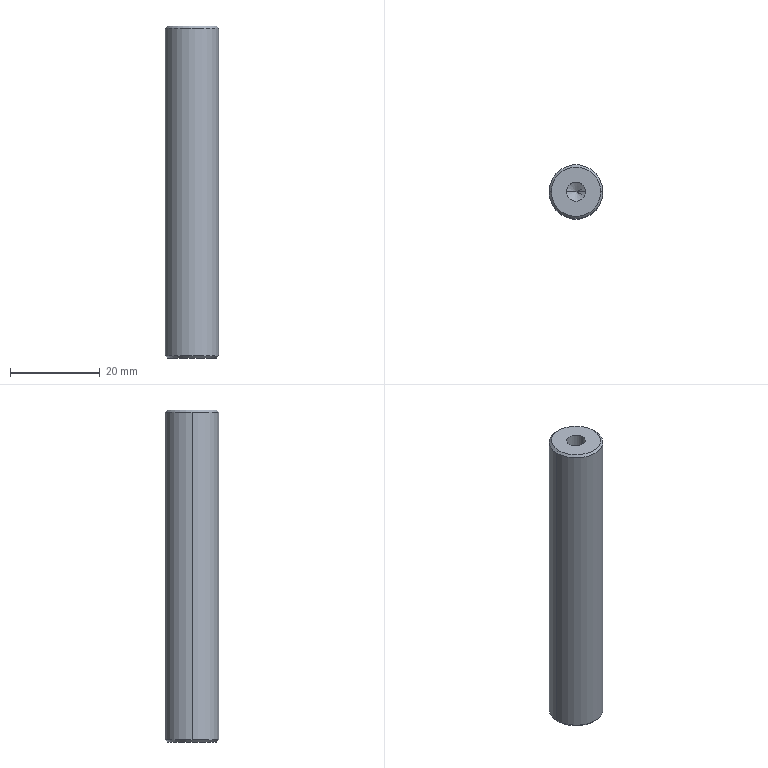Component | SolidWorks | J-028-1 | 1 solid | 12 faces | box 12 x 12 x 74 mm | volume 8182 mm3 | cone 6 | cylinder 4 | plane 2 | commonest cylinder face diameters 4.2 x2 12 x2 | material 45
build123d program:
from build123d import *

# Parameters (mm, degrees)
SKETCH1_R             = 6
BOSS_EXTRUDE1_DEPTH   = 74
CHAMFER1_SIZE         = 0.5
M5_TAPPED_HOLE1_D     = 4.2
M5_TAPPED_HOLE1_DEPTH = 12.4
M5_TAPPED_HOLE1_TIP   = 1.262


with BuildPart() as part:
    # Sketch1 → Boss-Extrude1 (new body)
    with BuildSketch(Plane(origin=(0, 0, 0), x_dir=(0, 0, -1), z_dir=(1, 0, 0))):
        Circle(SKETCH1_R)
    extrude(amount=BOSS_EXTRUDE1_DEPTH)

    # Chamfer1
    chamfer1_edges = [part.edges().sort_by_distance(p)[0] for p in [
        (0, 0, 6),
        (74, 0, 6),
    ]]
    chamfer(chamfer1_edges, length=CHAMFER1_SIZE)

    # M5 Tapped Hole1
    with Locations(Plane.ZY):
        with Locations((0, 0)):
            Hole(M5_TAPPED_HOLE1_D / 2, depth=M5_TAPPED_HOLE1_DEPTH)
            with Locations((0, 0, -(M5_TAPPED_HOLE1_DEPTH + M5_TAPPED_HOLE1_TIP / 2))):  # 118° drill point
                Cone(0, M5_TAPPED_HOLE1_D / 2, M5_TAPPED_HOLE1_TIP, mode=Mode.SUBTRACT)


solid = part.part

# Placed as in the assembly
solid = solid.moved(Location((95.325, 243.019, 264.731), (0, 90, 0)))
STEP:
#1=COLOUR_RGB('',0.7922,0.8196,0.9333);
#2=FILL_AREA_STYLE_COLOUR('',#1);
#3=FILL_AREA_STYLE('',(#2));
#4=SURFACE_STYLE_FILL_AREA(#3);
#5=SURFACE_SIDE_STYLE('',(#4));
#6=SURFACE_STYLE_USAGE(.BOTH.,#5);
#7=PRESENTATION_STYLE_ASSIGNMENT((#6));
#8=CARTESIAN_POINT('',(3.67,9.568,9.934));
#9=VERTEX_POINT('',#8);
#10=CARTESIAN_POINT('',(3.836,9.568,9.934));
#11=VERTEX_POINT('',#10);
#12=CARTESIAN_POINT('',(3.753,9.568,9.934));
#13=DIRECTION('',(0.,0.,1.));
#14=DIRECTION('',(1.,0.,0.));
#15=AXIS2_PLACEMENT_3D('',#12,#13,#14);
#16=CIRCLE('',#15,0.08268);
#17=EDGE_CURVE('',#9,#11,#16,.T.);
#18=ORIENTED_EDGE('',*,*,#17,.F.);
#19=CARTESIAN_POINT('',(3.67,9.568,10.422));
#20=VERTEX_POINT('',#19);
#21=CARTESIAN_POINT('',(3.67,9.568,10.422));
#22=DIRECTION('',(0.,0.,1.));
#23=VECTOR('',#22,39.37);
#24=LINE('',#21,#23);
#25=EDGE_CURVE('',#9,#20,#24,.T.);
#26=ORIENTED_EDGE('',*,*,#25,.T.);
#27=CARTESIAN_POINT('',(3.836,9.568,10.422));
#28=VERTEX_POINT('',#27);
#29=CARTESIAN_POINT('',(3.753,9.568,10.422));
#30=DIRECTION('',(0.,0.,1.));
#31=DIRECTION('',(1.,0.,0.));
#32=AXIS2_PLACEMENT_3D('',#29,#30,#31);
#33=CIRCLE('',#32,0.08268);
#34=EDGE_CURVE('',#20,#28,#33,.T.);
#35=ORIENTED_EDGE('',*,*,#34,.T.);
#36=CARTESIAN_POINT('',(3.836,9.568,10.422));
#37=DIRECTION('',(0.,0.,1.));
#38=VECTOR('',#37,39.37);
#39=LINE('',#36,#38);
#40=EDGE_CURVE('',#11,#28,#39,.T.);
#41=ORIENTED_EDGE('',*,*,#40,.F.);
#42=EDGE_LOOP('',(#18,#26,#35,#41));
#43=FACE_OUTER_BOUND('',#42,.T.);
#44=CARTESIAN_POINT('',(3.753,9.568,10.422));
#45=DIRECTION('',(0.,0.,1.));
#46=DIRECTION('',(1.,0.,0.));
#47=AXIS2_PLACEMENT_3D('',#44,#45,#46);
#48=CYLINDRICAL_SURFACE('',#47,0.08268);
#49=ADVANCED_FACE('',(#43),#48,.F.);
#50=CARTESIAN_POINT('',(3.753,9.568,9.885));
#51=VERTEX_POINT('',#50);
#52=CARTESIAN_POINT('',(3.836,9.568,9.934));
#53=DIRECTION('',(0.8572,0.,0.515));
#54=VECTOR('',#53,39.37);
#55=LINE('',#52,#54);
#56=EDGE_CURVE('',#51,#11,#55,.T.);
#57=ORIENTED_EDGE('',*,*,#56,.F.);
#58=CARTESIAN_POINT('',(3.67,9.568,9.934));
#59=DIRECTION('',(-0.8572,0.,0.515));
#60=VECTOR('',#59,39.37);
#61=LINE('',#58,#60);
#62=EDGE_CURVE('',#51,#9,#61,.T.);
#63=ORIENTED_EDGE('',*,*,#62,.T.);
#64=ORIENTED_EDGE('',*,*,#17,.T.);
#65=EDGE_LOOP('',(#57,#63,#64));
#66=FACE_OUTER_BOUND('',#65,.T.);
#67=CARTESIAN_POINT('',(3.753,9.568,9.934));
#68=DIRECTION('',(0.,0.,1.));
#69=DIRECTION('',(1.,0.,0.));
#70=AXIS2_PLACEMENT_3D('',#67,#68,#69);
#71=CONICAL_SURFACE('',#70,0.08268,1.03);
#72=ADVANCED_FACE('',(#66),#71,.F.);
#73=CARTESIAN_POINT('',(3.969,9.568,10.422));
#74=VERTEX_POINT('',#73);
#75=CARTESIAN_POINT('',(3.536,9.568,10.422));
#76=VERTEX_POINT('',#75);
#77=CARTESIAN_POINT('',(3.753,9.568,10.422));
#78=DIRECTION('',(0.,0.,1.));
#79=DIRECTION('',(-1.,0.,0.));
#80=AXIS2_PLACEMENT_3D('',#77,#78,#79);
#81=CIRCLE('',#80,0.2165);
#82=EDGE_CURVE('',#74,#76,#81,.T.);
#83=ORIENTED_EDGE('',*,*,#82,.F.);
#84=CARTESIAN_POINT('',(3.989,9.568,10.403));
#85=VERTEX_POINT('',#84);
#86=CARTESIAN_POINT('',(3.989,9.568,10.403));
#87=DIRECTION('',(0.7071,0.,-0.7071));
#88=VECTOR('',#87,39.37);
#89=LINE('',#86,#88);
#90=EDGE_CURVE('',#74,#85,#89,.T.);
#91=ORIENTED_EDGE('',*,*,#90,.T.);
#92=CARTESIAN_POINT('',(3.517,9.568,10.403));
#93=VERTEX_POINT('',#92);
#94=CARTESIAN_POINT('',(3.753,9.568,10.403));
#95=DIRECTION('',(0.,0.,-1.));
#96=DIRECTION('',(-1.,0.,0.));
#97=AXIS2_PLACEMENT_3D('',#94,#95,#96);
#98=CIRCLE('',#97,0.2362);
#99=EDGE_CURVE('',#93,#85,#98,.T.);
#100=ORIENTED_EDGE('',*,*,#99,.F.);
#101=CARTESIAN_POINT('',(3.517,9.568,10.403));
#102=DIRECTION('',(-0.7071,0.,-0.7071));
#103=VECTOR('',#102,39.37);
#104=LINE('',#101,#103);
#105=EDGE_CURVE('',#76,#93,#104,.T.);
#106=ORIENTED_EDGE('',*,*,#105,.F.);
#107=EDGE_LOOP('',(#83,#91,#100,#106));
#108=FACE_OUTER_BOUND('',#107,.T.);
#109=CARTESIAN_POINT('',(3.753,9.568,10.403));
#110=DIRECTION('',(0.,0.,-1.));
#111=DIRECTION('',(-1.,0.,0.));
#112=AXIS2_PLACEMENT_3D('',#109,#110,#111);
#113=CONICAL_SURFACE('',#112,0.2362,0.7854);
#114=ADVANCED_FACE('',(#108),#113,.T.);
#115=CARTESIAN_POINT('',(3.536,9.568,7.509));
#116=VERTEX_POINT('',#115);
#117=CARTESIAN_POINT('',(3.969,9.568,7.509));
#118=VERTEX_POINT('',#117);
#119=CARTESIAN_POINT('',(3.753,9.568,7.509));
#120=DIRECTION('',(0.,0.,-1.));
#121=DIRECTION('',(-1.,0.,0.));
#122=AXIS2_PLACEMENT_3D('',#119,#120,#121);
#123=CIRCLE('',#122,0.2165);
#124=EDGE_CURVE('',#116,#118,#123,.T.);
#125=ORIENTED_EDGE('',*,*,#124,.F.);
#126=CARTESIAN_POINT('',(3.517,9.568,7.529));
#127=VERTEX_POINT('',#126);
#128=CARTESIAN_POINT('',(3.536,9.568,7.509));
#129=DIRECTION('',(-0.7071,0.,0.7071));
#130=VECTOR('',#129,39.37);
#131=LINE('',#128,#130);
#132=EDGE_CURVE('',#116,#127,#131,.T.);
#133=ORIENTED_EDGE('',*,*,#132,.T.);
#134=CARTESIAN_POINT('',(3.989,9.568,7.529));
#135=VERTEX_POINT('',#134);
#136=CARTESIAN_POINT('',(3.753,9.568,7.529));
#137=DIRECTION('',(0.,0.,1.));
#138=DIRECTION('',(-1.,0.,0.));
#139=AXIS2_PLACEMENT_3D('',#136,#137,#138);
#140=CIRCLE('',#139,0.2362);
#141=EDGE_CURVE('',#135,#127,#140,.T.);
#142=ORIENTED_EDGE('',*,*,#141,.F.);
#143=CARTESIAN_POINT('',(3.969,9.568,7.509));
#144=DIRECTION('',(0.7071,0.,0.7071));
#145=VECTOR('',#144,39.37);
#146=LINE('',#143,#145);
#147=EDGE_CURVE('',#118,#135,#146,.T.);
#148=ORIENTED_EDGE('',*,*,#147,.F.);
#149=EDGE_LOOP('',(#125,#133,#142,#148));
#150=FACE_OUTER_BOUND('',#149,.T.);
#151=CARTESIAN_POINT('',(3.753,9.568,7.509));
#152=DIRECTION('',(0.,0.,1.));
#153=DIRECTION('',(1.,0.,0.));
#154=AXIS2_PLACEMENT_3D('',#151,#152,#153);
#155=CONICAL_SURFACE('',#154,0.2165,0.7854);
#156=ADVANCED_FACE('',(#150),#155,.T.);
#157=ORIENTED_EDGE('',*,*,#141,.T.);
#158=CARTESIAN_POINT('',(3.517,9.568,7.509));
#159=DIRECTION('',(0.,0.,1.));
#160=VECTOR('',#159,39.37);
#161=LINE('',#158,#160);
#162=EDGE_CURVE('',#127,#93,#161,.T.);
#163=ORIENTED_EDGE('',*,*,#162,.T.);
#164=ORIENTED_EDGE('',*,*,#99,.T.);
#165=CARTESIAN_POINT('',(3.989,9.568,7.509));
#166=DIRECTION('',(0.,0.,1.));
#167=VECTOR('',#166,39.37);
#168=LINE('',#165,#167);
#169=EDGE_CURVE('',#135,#85,#168,.T.);
#170=ORIENTED_EDGE('',*,*,#169,.F.);
#171=EDGE_LOOP('',(#157,#163,#164,#170));
#172=FACE_OUTER_BOUND('',#171,.T.);
#173=CARTESIAN_POINT('',(3.753,9.568,7.509));
#174=DIRECTION('',(0.,0.,1.));
#175=DIRECTION('',(1.,0.,0.));
#176=AXIS2_PLACEMENT_3D('',#173,#174,#175);
#177=CYLINDRICAL_SURFACE('',#176,0.2362);
#178=ADVANCED_FACE('',(#172),#177,.T.);
#179=ORIENTED_EDGE('',*,*,#162,.F.);
#180=CARTESIAN_POINT('',(3.753,9.568,7.529));
#181=DIRECTION('',(0.,0.,1.));
#182=DIRECTION('',(-1.,0.,0.));
#183=AXIS2_PLACEMENT_3D('',#180,#181,#182);
#184=CIRCLE('',#183,0.2362);
#185=EDGE_CURVE('',#127,#135,#184,.T.);
#186=ORIENTED_EDGE('',*,*,#185,.T.);
#187=ORIENTED_EDGE('',*,*,#169,.T.);
#188=CARTESIAN_POINT('',(3.753,9.568,10.403));
#189=DIRECTION('',(0.,0.,-1.));
#190=DIRECTION('',(-1.,0.,0.));
#191=AXIS2_PLACEMENT_3D('',#188,#189,#190);
#192=CIRCLE('',#191,0.2362);
#193=EDGE_CURVE('',#85,#93,#192,.T.);
#194=ORIENTED_EDGE('',*,*,#193,.T.);
#195=EDGE_LOOP('',(#179,#186,#187,#194));
#196=FACE_OUTER_BOUND('',#195,.T.);
#197=CARTESIAN_POINT('',(3.753,9.568,7.509));
#198=DIRECTION('',(0.,0.,1.));
#199=DIRECTION('',(1.,0.,0.));
#200=AXIS2_PLACEMENT_3D('',#197,#198,#199);
#201=CYLINDRICAL_SURFACE('',#200,0.2362);
#202=ADVANCED_FACE('',(#196),#201,.T.);
#203=CARTESIAN_POINT('',(3.753,9.568,7.509));
#204=DIRECTION('',(0.,0.,-1.));
#205=DIRECTION('',(-1.,0.,0.));
#206=AXIS2_PLACEMENT_3D('',#203,#204,#205);
#207=CIRCLE('',#206,0.2165);
#208=EDGE_CURVE('',#118,#116,#207,.T.);
#209=ORIENTED_EDGE('',*,*,#208,.T.);
#210=ORIENTED_EDGE('',*,*,#124,.T.);
#211=EDGE_LOOP('',(#209,#210));
#212=FACE_OUTER_BOUND('',#211,.T.);
#213=CARTESIAN_POINT('',(3.753,9.568,7.509));
#214=DIRECTION('',(0.,0.,-1.));
#215=DIRECTION('',(-1.,0.,0.));
#216=AXIS2_PLACEMENT_3D('',#213,#214,#215);
#217=PLANE('',#216);
#218=ADVANCED_FACE('',(#212),#217,.T.);
#219=CARTESIAN_POINT('',(3.753,9.568,10.422));
#220=DIRECTION('',(0.,0.,1.));
#221=DIRECTION('',(1.,0.,0.));
#222=AXIS2_PLACEMENT_3D('',#219,#220,#221);
#223=CIRCLE('',#222,0.08268);
#224=EDGE_CURVE('',#28,#20,#223,.T.);
#225=ORIENTED_EDGE('',*,*,#224,.F.);
#226=ORIENTED_EDGE('',*,*,#34,.F.);
#227=EDGE_LOOP('',(#225,#226));
#228=FACE_BOUND('',#227,.T.);
#229=CARTESIAN_POINT('',(3.753,9.568,10.422));
#230=DIRECTION('',(0.,0.,1.));
#231=DIRECTION('',(-1.,0.,0.));
#232=AXIS2_PLACEMENT_3D('',#229,#230,#231);
#233=CIRCLE('',#232,0.2165);
#234=EDGE_CURVE('',#76,#74,#233,.T.);
#235=ORIENTED_EDGE('',*,*,#234,.T.);
#236=ORIENTED_EDGE('',*,*,#82,.T.);
#237=EDGE_LOOP('',(#235,#236));
#238=FACE_OUTER_BOUND('',#237,.T.);
#239=CARTESIAN_POINT('',(3.753,9.568,10.422));
#240=DIRECTION('',(0.,0.,-1.));
#241=DIRECTION('',(-1.,0.,0.));
#242=AXIS2_PLACEMENT_3D('',#239,#240,#241);
#243=PLANE('',#242);
#244=ADVANCED_FACE('',(#228,#238),#243,.F.);
#245=ORIENTED_EDGE('',*,*,#132,.F.);
#246=ORIENTED_EDGE('',*,*,#208,.F.);
#247=ORIENTED_EDGE('',*,*,#147,.T.);
#248=ORIENTED_EDGE('',*,*,#185,.F.);
#249=EDGE_LOOP('',(#245,#246,#247,#248));
#250=FACE_OUTER_BOUND('',#249,.T.);
#251=CARTESIAN_POINT('',(3.753,9.568,7.509));
#252=DIRECTION('',(0.,0.,1.));
#253=DIRECTION('',(1.,0.,0.));
#254=AXIS2_PLACEMENT_3D('',#251,#252,#253);
#255=CONICAL_SURFACE('',#254,0.2165,0.7854);
#256=ADVANCED_FACE('',(#250),#255,.T.);
#257=ORIENTED_EDGE('',*,*,#90,.F.);
#258=ORIENTED_EDGE('',*,*,#234,.F.);
#259=ORIENTED_EDGE('',*,*,#105,.T.);
#260=ORIENTED_EDGE('',*,*,#193,.F.);
#261=EDGE_LOOP('',(#257,#258,#259,#260));
#262=FACE_OUTER_BOUND('',#261,.T.);
#263=CARTESIAN_POINT('',(3.753,9.568,10.403));
#264=DIRECTION('',(0.,0.,-1.));
#265=DIRECTION('',(-1.,0.,0.));
#266=AXIS2_PLACEMENT_3D('',#263,#264,#265);
#267=CONICAL_SURFACE('',#266,0.2362,0.7854);
#268=ADVANCED_FACE('',(#262),#267,.T.);
#269=ORIENTED_EDGE('',*,*,#62,.F.);
#270=ORIENTED_EDGE('',*,*,#56,.T.);
#271=CARTESIAN_POINT('',(3.753,9.568,9.934));
#272=DIRECTION('',(0.,0.,1.));
#273=DIRECTION('',(1.,0.,0.));
#274=AXIS2_PLACEMENT_3D('',#271,#272,#273);
#275=CIRCLE('',#274,0.08268);
#276=EDGE_CURVE('',#11,#9,#275,.T.);
#277=ORIENTED_EDGE('',*,*,#276,.T.);
#278=EDGE_LOOP('',(#269,#270,#277));
#279=FACE_OUTER_BOUND('',#278,.T.);
#280=CARTESIAN_POINT('',(3.753,9.568,9.934));
#281=DIRECTION('',(0.,0.,1.));
#282=DIRECTION('',(1.,0.,0.));
#283=AXIS2_PLACEMENT_3D('',#280,#281,#282);
#284=CONICAL_SURFACE('',#283,0.08268,1.03);
#285=ADVANCED_FACE('',(#279),#284,.F.);
#286=ORIENTED_EDGE('',*,*,#25,.F.);
#287=ORIENTED_EDGE('',*,*,#276,.F.);
#288=ORIENTED_EDGE('',*,*,#40,.T.);
#289=ORIENTED_EDGE('',*,*,#224,.T.);
#290=EDGE_LOOP('',(#286,#287,#288,#289));
#291=FACE_OUTER_BOUND('',#290,.T.);
#292=CARTESIAN_POINT('',(3.753,9.568,10.422));
#293=DIRECTION('',(0.,0.,1.));
#294=DIRECTION('',(1.,0.,0.));
#295=AXIS2_PLACEMENT_3D('',#292,#293,#294);
#296=CYLINDRICAL_SURFACE('',#295,0.08268);
#297=ADVANCED_FACE('',(#291),#296,.F.);
#298=CLOSED_SHELL('',(#49,#72,#114,#156,#178,#202,#218,#244,#256,#268,#285,#297));
#299=MANIFOLD_SOLID_BREP('',#298);
#300=STYLED_ITEM('',(#7),#299);
#301=(LENGTH_UNIT()NAMED_UNIT(*)SI_UNIT($,.METRE.));
#302=LENGTH_MEASURE_WITH_UNIT(LENGTH_MEASURE(0.0254),#301);
#303=DIMENSIONAL_EXPONENTS(1.,0.,0.,0.,0.,0.,0.);
#304=(CONVERSION_BASED_UNIT('',#302)LENGTH_UNIT()NAMED_UNIT(#303));
#305=UNCERTAINTY_MEASURE_WITH_UNIT(LENGTH_MEASURE(0.00001),#304,'','');
#306=(NAMED_UNIT(*)PLANE_ANGLE_UNIT()SI_UNIT($,.RADIAN.));
#307=(NAMED_UNIT(*)SI_UNIT($,.STERADIAN.)SOLID_ANGLE_UNIT());
#308=(GEOMETRIC_REPRESENTATION_CONTEXT(3)GLOBAL_UNCERTAINTY_ASSIGNED_CONTEXT((#305))GLOBAL_UNIT_ASSIGNED_CONTEXT((#304,#306,#307))REPRESENTATION_CONTEXT('',''));
#309=MECHANICAL_DESIGN_GEOMETRIC_PRESENTATION_REPRESENTATION('',(#300),#308);
#310=PRESENTATION_LAYER_ASSIGNMENT('','',(#300));
#311=CARTESIAN_POINT('',(0.,0.,0.));
#312=DIRECTION('',(0.,0.,1.));
#313=DIRECTION('',(1.,0.,0.));
#314=AXIS2_PLACEMENT_3D('',#311,#312,#313);
#315=(LENGTH_UNIT()NAMED_UNIT(*)SI_UNIT($,.METRE.));
#316=LENGTH_MEASURE_WITH_UNIT(LENGTH_MEASURE(0.0254),#315);
#317=DIMENSIONAL_EXPONENTS(1.,0.,0.,0.,0.,0.,0.);
#318=(CONVERSION_BASED_UNIT('',#316)LENGTH_UNIT()NAMED_UNIT(#317));
#319=UNCERTAINTY_MEASURE_WITH_UNIT(LENGTH_MEASURE(0.00001),#318,'','');
#320=(NAMED_UNIT(*)PLANE_ANGLE_UNIT()SI_UNIT($,.RADIAN.));
#321=(NAMED_UNIT(*)SI_UNIT($,.STERADIAN.)SOLID_ANGLE_UNIT());
#322=(GEOMETRIC_REPRESENTATION_CONTEXT(3)GLOBAL_UNCERTAINTY_ASSIGNED_CONTEXT((#319))GLOBAL_UNIT_ASSIGNED_CONTEXT((#318,#320,#321))REPRESENTATION_CONTEXT('',''));
#323=ADVANCED_BREP_SHAPE_REPRESENTATION('',(#299,#314),#322);